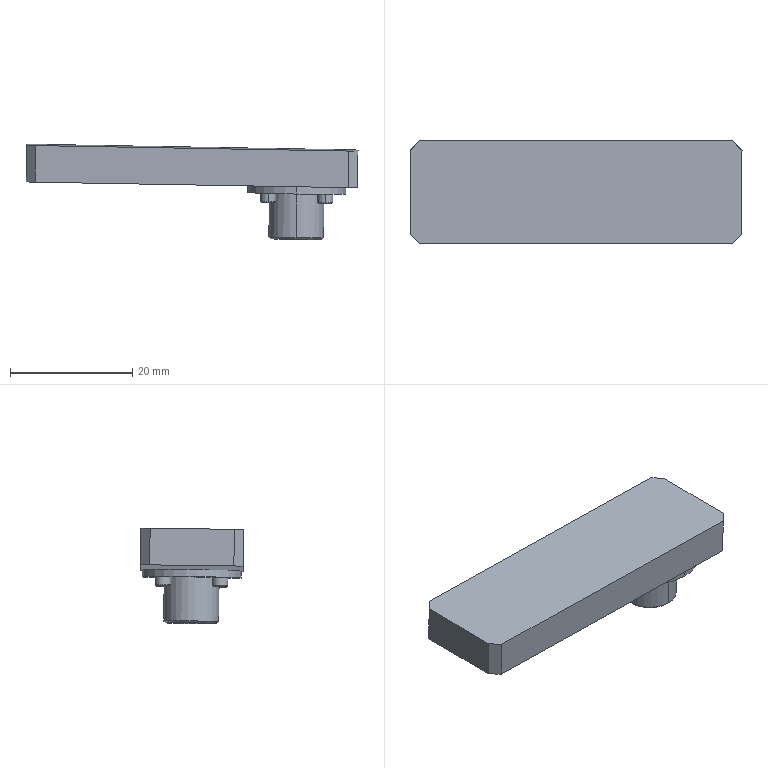Component | SolidWorks | 00-VacuumSuctionCupAssembly-1_07-Busbar-1 | 1 solid | 71 faces | box 54.4 x 16.87 x 15.65 mm | volume 5998 mm3 | plane 45 | cylinder 14 | cone 12 | commonest cylinder face diameters 2.496 x8 5.308 x2 9 x2 16.2 x2
build123d program:
from build123d import *

# Parameters (mm, degrees)
SKETCH1_W           = 181
SKETCH1_H           = 56
BOSS_EXTRUDE1_DEPTH = 20
SKETCH2_R           = 27
BOSS_EXTRUDE2_DEPTH = 4
SKETCH3_R           = 15
BOSS_EXTRUDE3_DEPTH = 25
SKETCH4_R           = 4.16
BOSS_EXTRUDE4_DEPTH = 5
CUT_EXTRUDE1_DEPTH  = 2
SKETCH6_R           = 4.16
BOSS_EXTRUDE5_DEPTH = 5
CUT_EXTRUDE2_DEPTH  = 2
SKETCH8_R           = 4.16
BOSS_EXTRUDE6_DEPTH = 5
CUT_EXTRUDE3_DEPTH  = 2
SKETCH10_R          = 4.16
BOSS_EXTRUDE7_DEPTH = 5
CUT_EXTRUDE4_DEPTH  = 2
CHAMFER1_SIZE       = 1
CHAMFER2_SIZE       = 5
CHAMFER3_SIZE       = 0.5
SCALE1_SCALE        = 0.3


with BuildPart() as part:
    # Sketch1 → Boss-Extrude1 (new body)
    with BuildSketch(Plane(origin=(0, 20, 0), x_dir=(1, 0, 0), z_dir=(0, 1, 0))):
        with Locations((90.5, 0)):
            Rectangle(SKETCH1_W, SKETCH1_H)
    extrude(amount=-BOSS_EXTRUDE1_DEPTH)

    # Sketch2 → Boss-Extrude2 (add)
    with BuildSketch(Plane(origin=(0, 20, 0), x_dir=(-1, 0, 0), z_dir=(0, 1, 0))):
        with Locations(Location((-33, 0, 0), (0, 0, 90))):
            Circle(SKETCH2_R)
    extrude(amount=BOSS_EXTRUDE2_DEPTH)

    # Sketch3 → Boss-Extrude3 (add)
    with BuildSketch(Plane(origin=(0, 24, 0), x_dir=(-1, 0, 0), z_dir=(0, 1, 0))):
        with Locations(Location((-33, 0, 0), (0, 0, 90))):
            Circle(SKETCH3_R)
    extrude(amount=BOSS_EXTRUDE3_DEPTH)

    # Sketch4 → Boss-Extrude4 (add)
    with BuildSketch(Plane(origin=(0, 24, 0), x_dir=(-1, 0, 0), z_dir=(0, 1, 0))):
        with Locations(Location((-17.444, -15.556, 0), (0, 0, 90))):
            Circle(SKETCH4_R)
    extrude(amount=BOSS_EXTRUDE4_DEPTH)

    # Sketch5 → Cut-Extrude1 (cut)
    with BuildSketch(Plane(origin=(0, 29, 0), x_dir=(-1, 0, 0), z_dir=(0, 1, 0))):
        Polygon((-17.444, -17.866), (-15.444, -16.711), (-15.444, -14.402), (-17.444, -13.247), (-19.444, -14.402), (-19.444, -16.711), align=None)
    extrude(amount=-CUT_EXTRUDE1_DEPTH, mode=Mode.SUBTRACT)

    # Sketch6 → Boss-Extrude5 (add)
    with BuildSketch(Plane(origin=(0, 24, 0), x_dir=(-1, 0, 0), z_dir=(0, 1, 0))):
        with Locations(Location((-48.556, -15.556, 0), (0, 0, 90))):
            Circle(SKETCH6_R)
    extrude(amount=BOSS_EXTRUDE5_DEPTH)

    # Sketch7 → Cut-Extrude2 (cut)
    with BuildSketch(Plane(origin=(0, 29, 0), x_dir=(-1, 0, 0), z_dir=(0, 1, 0))):
        Polygon((-48.556, -17.866), (-46.556, -16.711), (-46.556, -14.402), (-48.556, -13.247), (-50.556, -14.402), (-50.556, -16.711), align=None)
    extrude(amount=-CUT_EXTRUDE2_DEPTH, mode=Mode.SUBTRACT)

    # Sketch8 → Boss-Extrude6 (add)
    with BuildSketch(Plane(origin=(0, 24, 0), x_dir=(-1, 0, 0), z_dir=(0, 1, 0))):
        with Locations(Location((-48.556, 15.556, 0), (0, 0, 90))):
            Circle(SKETCH8_R)
    extrude(amount=BOSS_EXTRUDE6_DEPTH)

    # Sketch9 → Cut-Extrude3 (cut)
    with BuildSketch(Plane(origin=(0, 29, 0), x_dir=(-1, 0, 0), z_dir=(0, 1, 0))):
        Polygon((-48.556, 13.247), (-46.556, 14.402), (-46.556, 16.711), (-48.556, 17.866), (-50.556, 16.711), (-50.556, 14.402), align=None)
    extrude(amount=-CUT_EXTRUDE3_DEPTH, mode=Mode.SUBTRACT)

    # Sketch10 → Boss-Extrude7 (add)
    with BuildSketch(Plane(origin=(0, 24, 0), x_dir=(-1, 0, 0), z_dir=(0, 1, 0))):
        with Locations(Location((-17.444, 15.556, 0), (0, 0, 90))):
            Circle(SKETCH10_R)
    extrude(amount=BOSS_EXTRUDE7_DEPTH)

    # Sketch11 → Cut-Extrude4 (cut)
    with BuildSketch(Plane(origin=(0, 29, 0), x_dir=(-1, 0, 0), z_dir=(0, 1, 0))):
        Polygon((-17.444, 13.247), (-15.444, 14.402), (-15.444, 16.711), (-17.444, 17.866), (-19.444, 16.711), (-19.444, 14.402), align=None)
    extrude(amount=-CUT_EXTRUDE4_DEPTH, mode=Mode.SUBTRACT)

    # Sketch12 → Conical Countersunk Hole for M16 Flat He (revolve, cut)
    with BuildSketch(Plane(origin=(33, 49, 0), x_dir=(0, 0, 1), z_dir=(1, 0, 0))):
        Polygon((0, 0), (0, 29), (8.847, 29), (8.847, 15), (9.316, 0), align=None)
    revolve(axis=Axis((33, 55.35, 0), (0, -1, 0)), mode=Mode.SUBTRACT)

    # Chamfer1
    chamfer1_edges = [part.edges().sort_by_distance(p)[0] for p in [
        (33, 49, -15),
    ]]
    chamfer(chamfer1_edges, length=CHAMFER1_SIZE)

    # Chamfer2
    chamfer2_edges = [part.edges().sort_by_distance(p)[0] for p in [
        (181, 10, -28),
        (181, 10, 28),
        (0, 10, 28),
        (0, 10, -28),
    ]]
    chamfer(chamfer2_edges, length=CHAMFER2_SIZE)

    # Chamfer3
    chamfer3_edges = [part.edges().sort_by_distance(p)[0] for p in [
        (17.444, 29, -19.716),
        (48.556, 29, -19.716),
        (48.556, 29, 11.396),
        (17.444, 29, 11.396),
    ]]
    chamfer(chamfer3_edges, length=CHAMFER3_SIZE)


with BuildPart() as part_1:
    # Scale1: scaled about (85.214, 11.849, 0)
    add(part.part.scale(SCALE1_SCALE).moved(Location((59.65, 8.294, 0))))


solid = part_1.part

# Placed as in the assembly
solid = solid.moved(Location((128.135, 133.544, 53.614), (90.721, -0.01259, 179)))